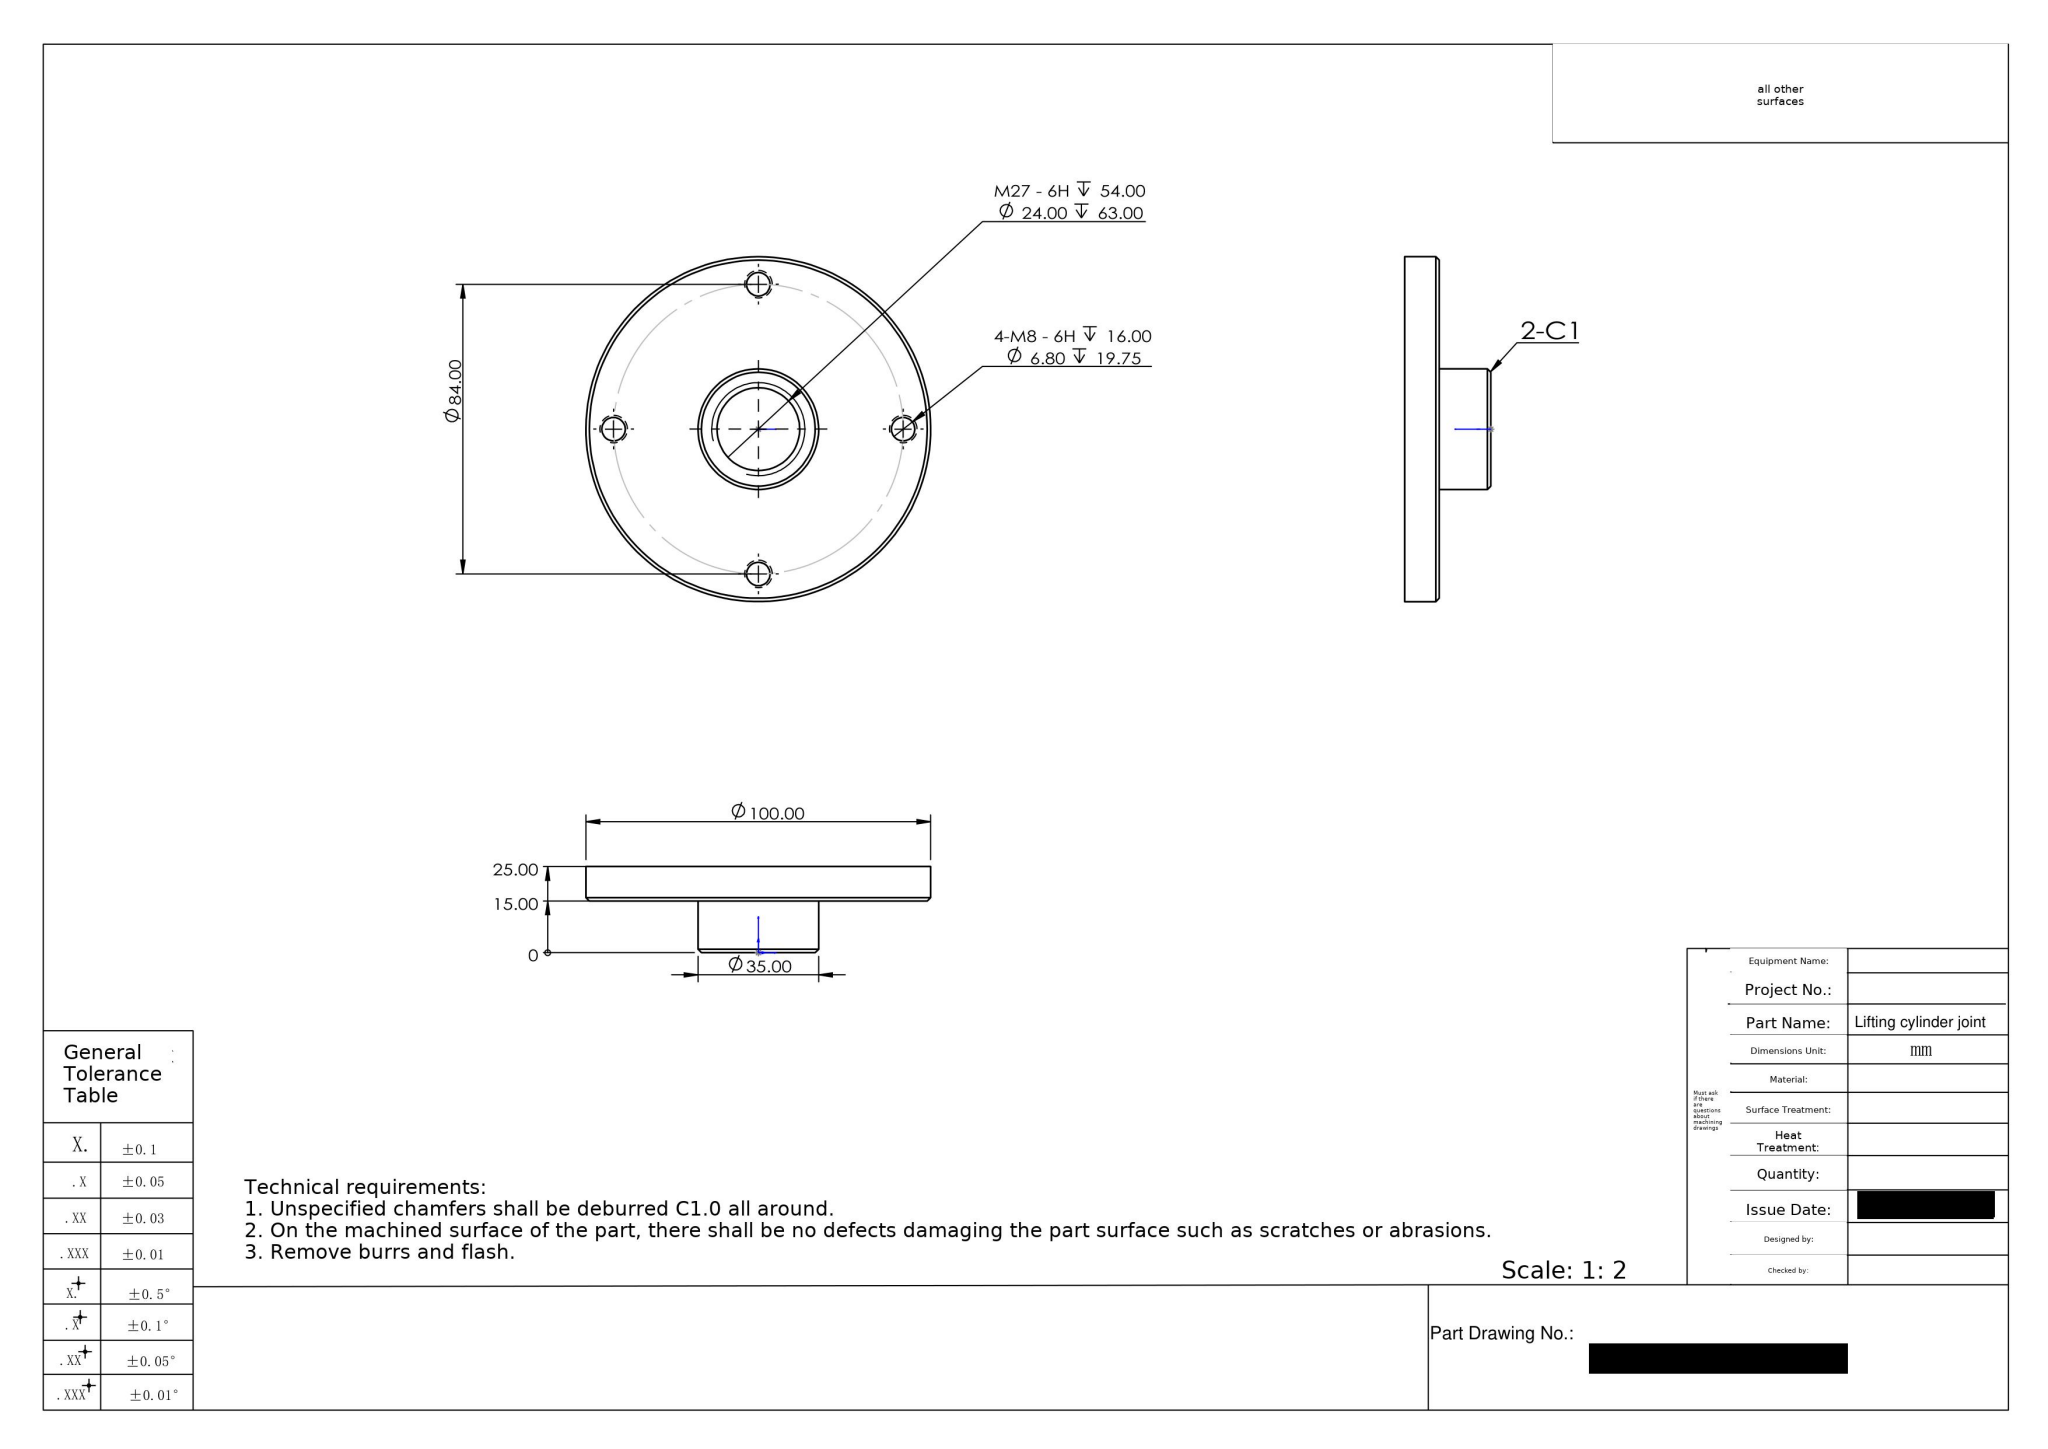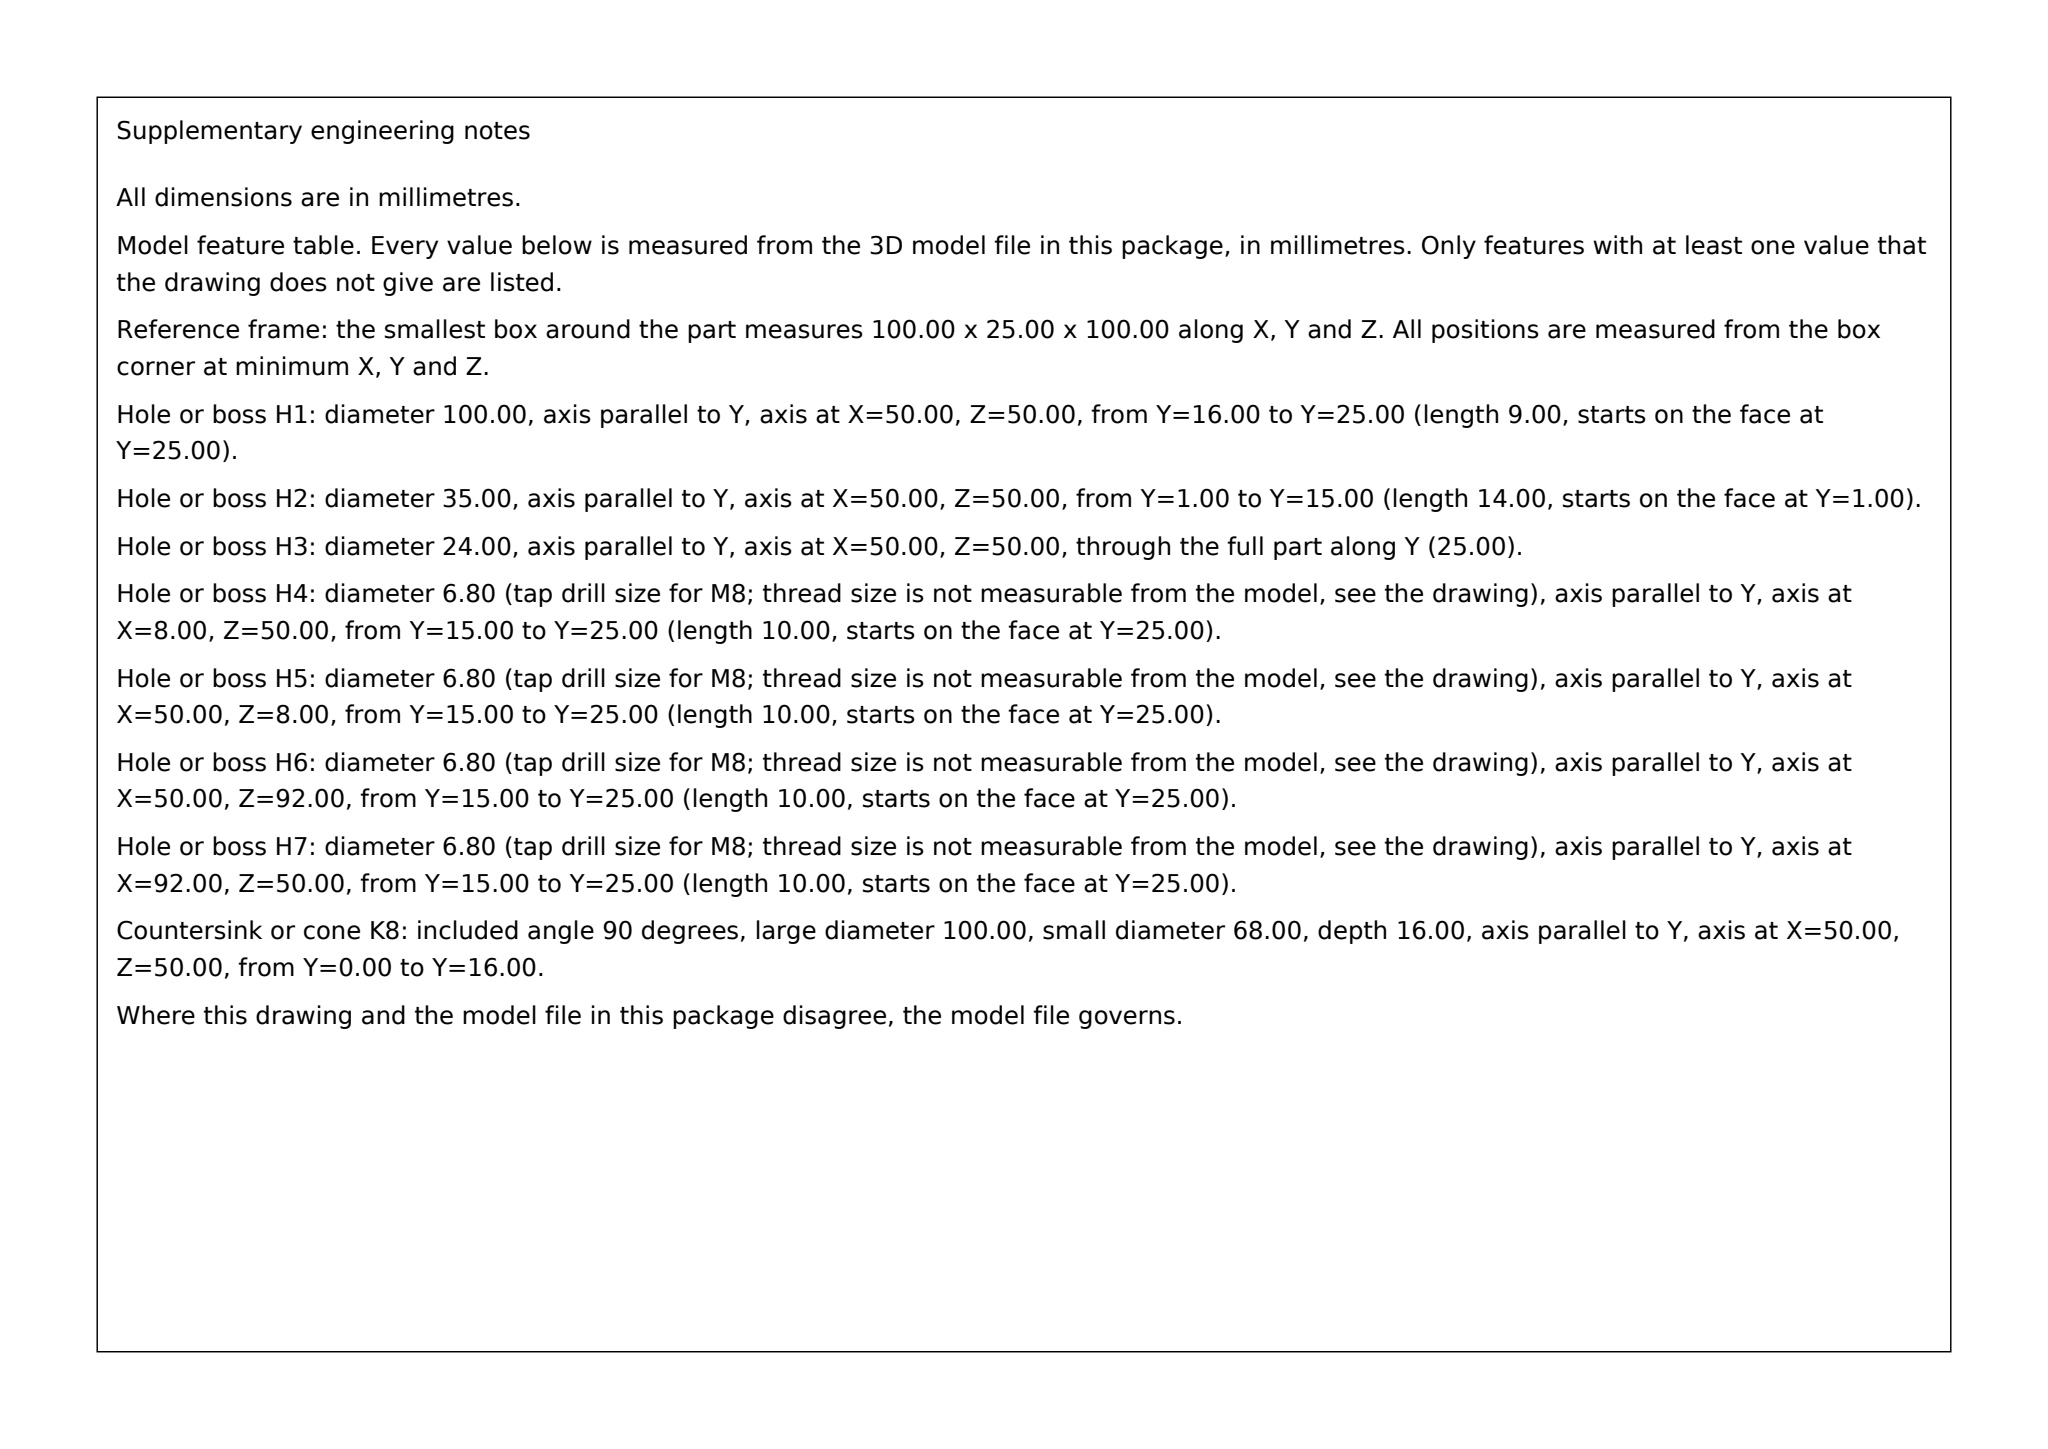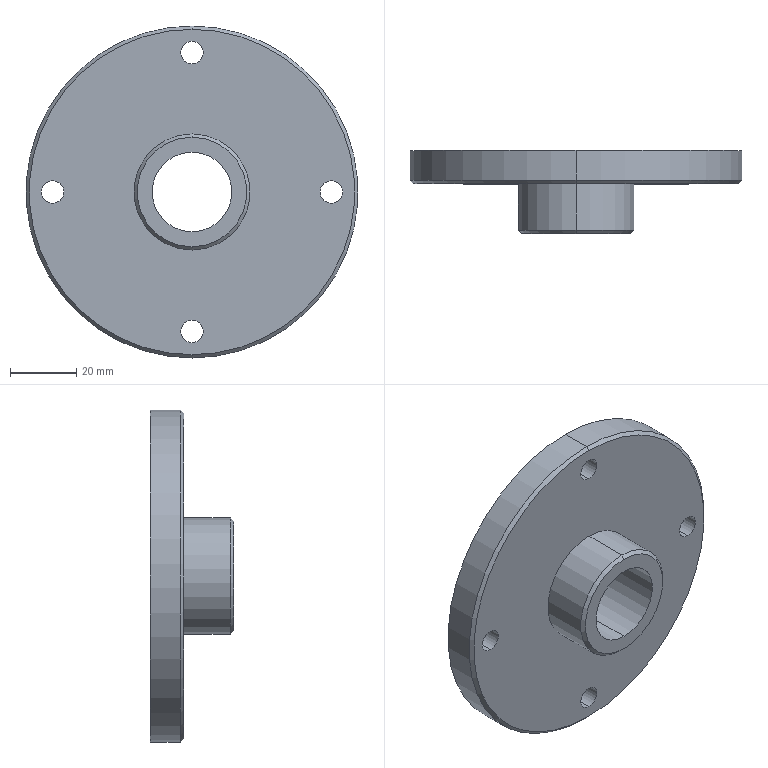Part | SolidWorks | mm | 1 solid | 21 faces | box 100 x 25 x 100 mm | volume 79999 mm3 | cylinder 14 | cone 4 | plane 3 | commonest cylinder face diameters 6.8 x8 24 x2 100 x2 35 x2
build123d program:
from build123d import *

# Parameters (mm, degrees)
SKETCH1_R              = 17.5
BOSS_EXTRUDE1_DEPTH    = 15
SKETCH2_R              = 50
BOSS_EXTRUDE2_DEPTH    = 10
M27_TAPPED_HOLE1_D     = 24
M27_TAPPED_HOLE1_DEPTH = 63
M27_TAPPED_HOLE1_TIP   = 7.21
M8_TAPPED_HOLE1_D      = 6.8
M8_TAPPED_HOLE1_DEPTH  = 19.75
M8_TAPPED_HOLE1_TIP    = 2.043
CHAMFER1_SIZE          = 1


with BuildPart() as part:
    # Sketch1 → Boss-Extrude1 (new body)
    with BuildSketch(Plane(origin=(0, 0, 0), x_dir=(1, 0, 0), z_dir=(0, 1, 0))):
        with Locations(Location((0, 0, 0), (0, 0, 270))):
            Circle(SKETCH1_R)
    extrude(amount=BOSS_EXTRUDE1_DEPTH)

    # Sketch2 → Boss-Extrude2 (add)
    with BuildSketch(Plane(origin=(0, 15, 0), x_dir=(1, 0, 0), z_dir=(0, 1, 0))):
        with Locations(Location((0, 0, 0), (0, 0, 270))):
            Circle(SKETCH2_R)
    extrude(amount=BOSS_EXTRUDE2_DEPTH)

    # M27 Tapped Hole1
    with Locations(Plane(origin=(0, 0, 0), x_dir=(-1, 0, 0), z_dir=(0, -1, 0))):
        with Locations((0, 0)):
            Hole(M27_TAPPED_HOLE1_D / 2, depth=M27_TAPPED_HOLE1_DEPTH)
            with Locations((0, 0, -(M27_TAPPED_HOLE1_DEPTH + M27_TAPPED_HOLE1_TIP / 2))):  # 118° drill point
                Cone(0, M27_TAPPED_HOLE1_D / 2, M27_TAPPED_HOLE1_TIP, mode=Mode.SUBTRACT)

    # M8 Tapped Hole1
    with Locations(Plane(origin=(0, 25, 0), x_dir=(1, 0, 0), z_dir=(0, 1, 0))):
        with Locations((0, 42), (42, 0), (0, -42), (-42, 0)):
            Hole(M8_TAPPED_HOLE1_D / 2, depth=M8_TAPPED_HOLE1_DEPTH)
            with Locations((0, 0, -(M8_TAPPED_HOLE1_DEPTH + M8_TAPPED_HOLE1_TIP / 2))):  # 118° drill point
                Cone(0, M8_TAPPED_HOLE1_D / 2, M8_TAPPED_HOLE1_TIP, mode=Mode.SUBTRACT)

    # Chamfer1
    chamfer1_edges = [part.edges().sort_by_distance(p)[0] for p in [
        (0, 0, -17.5),
        (0, 15, -50),
    ]]
    chamfer(chamfer1_edges, length=CHAMFER1_SIZE)


solid = part.part
STEP:
#1=CARTESIAN_POINT('',(0.,15.,-49.));
#2=VERTEX_POINT('',#1);
#3=CARTESIAN_POINT('',(0.,15.,49.));
#4=VERTEX_POINT('',#3);
#5=CARTESIAN_POINT('',(0.,15.,0.));
#6=DIRECTION('',(0.,-1.,0.));
#7=DIRECTION('',(0.,0.,1.));
#8=AXIS2_PLACEMENT_3D('',#5,#6,#7);
#9=CIRCLE('',#8,49.);
#10=EDGE_CURVE('',#2,#4,#9,.T.);
#11=ORIENTED_EDGE('',*,*,#10,.F.);
#12=CARTESIAN_POINT('',(0.,16.,-50.));
#13=VERTEX_POINT('',#12);
#14=CARTESIAN_POINT('',(0.,16.,-50.));
#15=DIRECTION('',(0.,0.7071,-0.7071));
#16=VECTOR('',#15,1000.);
#17=LINE('',#14,#16);
#18=EDGE_CURVE('',#2,#13,#17,.T.);
#19=ORIENTED_EDGE('',*,*,#18,.T.);
#20=CARTESIAN_POINT('',(0.,16.,50.));
#21=VERTEX_POINT('',#20);
#22=CARTESIAN_POINT('',(0.,16.,0.));
#23=DIRECTION('',(0.,1.,0.));
#24=DIRECTION('',(0.,0.,1.));
#25=AXIS2_PLACEMENT_3D('',#22,#23,#24);
#26=CIRCLE('',#25,50.);
#27=EDGE_CURVE('',#21,#13,#26,.T.);
#28=ORIENTED_EDGE('',*,*,#27,.F.);
#29=CARTESIAN_POINT('',(0.,16.,50.));
#30=DIRECTION('',(0.,0.7071,0.7071));
#31=VECTOR('',#30,1000.);
#32=LINE('',#29,#31);
#33=EDGE_CURVE('',#4,#21,#32,.T.);
#34=ORIENTED_EDGE('',*,*,#33,.F.);
#35=EDGE_LOOP('',(#11,#19,#28,#34));
#36=FACE_OUTER_BOUND('',#35,.T.);
#37=CARTESIAN_POINT('',(0.,16.,0.));
#38=DIRECTION('',(0.,1.,0.));
#39=DIRECTION('',(0.,0.,1.));
#40=AXIS2_PLACEMENT_3D('',#37,#38,#39);
#41=CONICAL_SURFACE('',#40,50.,0.7854);
#42=ADVANCED_FACE('',(#36),#41,.T.);
#43=CARTESIAN_POINT('',(0.,0.,-16.5));
#44=VERTEX_POINT('',#43);
#45=CARTESIAN_POINT('',(0.,0.,16.5));
#46=VERTEX_POINT('',#45);
#47=CARTESIAN_POINT('',(0.,0.,0.));
#48=DIRECTION('',(0.,-1.,0.));
#49=DIRECTION('',(0.,0.,1.));
#50=AXIS2_PLACEMENT_3D('',#47,#48,#49);
#51=CIRCLE('',#50,16.5);
#52=EDGE_CURVE('',#44,#46,#51,.T.);
#53=ORIENTED_EDGE('',*,*,#52,.F.);
#54=CARTESIAN_POINT('',(0.,1.,-17.5));
#55=VERTEX_POINT('',#54);
#56=CARTESIAN_POINT('',(0.,1.,-17.5));
#57=DIRECTION('',(0.,0.7071,-0.7071));
#58=VECTOR('',#57,1000.);
#59=LINE('',#56,#58);
#60=EDGE_CURVE('',#44,#55,#59,.T.);
#61=ORIENTED_EDGE('',*,*,#60,.T.);
#62=CARTESIAN_POINT('',(0.,1.,17.5));
#63=VERTEX_POINT('',#62);
#64=CARTESIAN_POINT('',(0.,1.,0.));
#65=DIRECTION('',(0.,1.,0.));
#66=DIRECTION('',(0.,0.,1.));
#67=AXIS2_PLACEMENT_3D('',#64,#65,#66);
#68=CIRCLE('',#67,17.5);
#69=EDGE_CURVE('',#63,#55,#68,.T.);
#70=ORIENTED_EDGE('',*,*,#69,.F.);
#71=CARTESIAN_POINT('',(0.,1.,17.5));
#72=DIRECTION('',(0.,0.7071,0.7071));
#73=VECTOR('',#72,1000.);
#74=LINE('',#71,#73);
#75=EDGE_CURVE('',#46,#63,#74,.T.);
#76=ORIENTED_EDGE('',*,*,#75,.F.);
#77=EDGE_LOOP('',(#53,#61,#70,#76));
#78=FACE_OUTER_BOUND('',#77,.T.);
#79=CARTESIAN_POINT('',(0.,1.,0.));
#80=DIRECTION('',(0.,1.,0.));
#81=DIRECTION('',(0.,0.,1.));
#82=AXIS2_PLACEMENT_3D('',#79,#80,#81);
#83=CONICAL_SURFACE('',#82,17.5,0.7854);
#84=ADVANCED_FACE('',(#78),#83,.T.);
#85=CARTESIAN_POINT('',(0.,15.,-45.4));
#86=VERTEX_POINT('',#85);
#87=CARTESIAN_POINT('',(0.,15.,-38.6));
#88=VERTEX_POINT('',#87);
#89=CARTESIAN_POINT('',(0.,15.,-42.));
#90=DIRECTION('',(0.,1.,0.));
#91=DIRECTION('',(0.,0.,1.));
#92=AXIS2_PLACEMENT_3D('',#89,#90,#91);
#93=CIRCLE('',#92,3.4);
#94=EDGE_CURVE('',#86,#88,#93,.T.);
#95=ORIENTED_EDGE('',*,*,#94,.F.);
#96=CARTESIAN_POINT('',(0.,25.,-45.4));
#97=VERTEX_POINT('',#96);
#98=CARTESIAN_POINT('',(0.,25.,-45.4));
#99=DIRECTION('',(0.,1.,0.));
#100=VECTOR('',#99,1000.);
#101=LINE('',#98,#100);
#102=EDGE_CURVE('',#86,#97,#101,.T.);
#103=ORIENTED_EDGE('',*,*,#102,.T.);
#104=CARTESIAN_POINT('',(0.,25.,-38.6));
#105=VERTEX_POINT('',#104);
#106=CARTESIAN_POINT('',(0.,25.,-42.));
#107=DIRECTION('',(0.,1.,0.));
#108=DIRECTION('',(0.,0.,1.));
#109=AXIS2_PLACEMENT_3D('',#106,#107,#108);
#110=CIRCLE('',#109,3.4);
#111=EDGE_CURVE('',#97,#105,#110,.T.);
#112=ORIENTED_EDGE('',*,*,#111,.T.);
#113=CARTESIAN_POINT('',(0.,25.,-38.6));
#114=DIRECTION('',(0.,1.,0.));
#115=VECTOR('',#114,1000.);
#116=LINE('',#113,#115);
#117=EDGE_CURVE('',#88,#105,#116,.T.);
#118=ORIENTED_EDGE('',*,*,#117,.F.);
#119=EDGE_LOOP('',(#95,#103,#112,#118));
#120=FACE_OUTER_BOUND('',#119,.T.);
#121=CARTESIAN_POINT('',(0.,25.,-42.));
#122=DIRECTION('',(0.,1.,0.));
#123=DIRECTION('',(0.,0.,1.));
#124=AXIS2_PLACEMENT_3D('',#121,#122,#123);
#125=CYLINDRICAL_SURFACE('',#124,3.4);
#126=ADVANCED_FACE('',(#120),#125,.F.);
#127=CARTESIAN_POINT('',(42.,15.,-3.4));
#128=VERTEX_POINT('',#127);
#129=CARTESIAN_POINT('',(42.,15.,3.4));
#130=VERTEX_POINT('',#129);
#131=CARTESIAN_POINT('',(42.,15.,0.));
#132=DIRECTION('',(0.,1.,0.));
#133=DIRECTION('',(0.,0.,1.));
#134=AXIS2_PLACEMENT_3D('',#131,#132,#133);
#135=CIRCLE('',#134,3.4);
#136=EDGE_CURVE('',#128,#130,#135,.T.);
#137=ORIENTED_EDGE('',*,*,#136,.F.);
#138=CARTESIAN_POINT('',(42.,25.,-3.4));
#139=VERTEX_POINT('',#138);
#140=CARTESIAN_POINT('',(42.,25.,-3.4));
#141=DIRECTION('',(0.,1.,0.));
#142=VECTOR('',#141,1000.);
#143=LINE('',#140,#142);
#144=EDGE_CURVE('',#128,#139,#143,.T.);
#145=ORIENTED_EDGE('',*,*,#144,.T.);
#146=CARTESIAN_POINT('',(42.,25.,3.4));
#147=VERTEX_POINT('',#146);
#148=CARTESIAN_POINT('',(42.,25.,0.));
#149=DIRECTION('',(0.,1.,0.));
#150=DIRECTION('',(0.,0.,1.));
#151=AXIS2_PLACEMENT_3D('',#148,#149,#150);
#152=CIRCLE('',#151,3.4);
#153=EDGE_CURVE('',#139,#147,#152,.T.);
#154=ORIENTED_EDGE('',*,*,#153,.T.);
#155=CARTESIAN_POINT('',(42.,25.,3.4));
#156=DIRECTION('',(0.,1.,0.));
#157=VECTOR('',#156,1000.);
#158=LINE('',#155,#157);
#159=EDGE_CURVE('',#130,#147,#158,.T.);
#160=ORIENTED_EDGE('',*,*,#159,.F.);
#161=EDGE_LOOP('',(#137,#145,#154,#160));
#162=FACE_OUTER_BOUND('',#161,.T.);
#163=CARTESIAN_POINT('',(42.,25.,0.));
#164=DIRECTION('',(0.,1.,0.));
#165=DIRECTION('',(0.,0.,1.));
#166=AXIS2_PLACEMENT_3D('',#163,#164,#165);
#167=CYLINDRICAL_SURFACE('',#166,3.4);
#168=ADVANCED_FACE('',(#162),#167,.F.);
#169=CARTESIAN_POINT('',(0.,15.,38.6));
#170=VERTEX_POINT('',#169);
#171=CARTESIAN_POINT('',(0.,15.,45.4));
#172=VERTEX_POINT('',#171);
#173=CARTESIAN_POINT('',(0.,15.,42.));
#174=DIRECTION('',(0.,1.,0.));
#175=DIRECTION('',(0.,0.,1.));
#176=AXIS2_PLACEMENT_3D('',#173,#174,#175);
#177=CIRCLE('',#176,3.4);
#178=EDGE_CURVE('',#170,#172,#177,.T.);
#179=ORIENTED_EDGE('',*,*,#178,.F.);
#180=CARTESIAN_POINT('',(0.,25.,38.6));
#181=VERTEX_POINT('',#180);
#182=CARTESIAN_POINT('',(0.,25.,38.6));
#183=DIRECTION('',(0.,1.,0.));
#184=VECTOR('',#183,1000.);
#185=LINE('',#182,#184);
#186=EDGE_CURVE('',#170,#181,#185,.T.);
#187=ORIENTED_EDGE('',*,*,#186,.T.);
#188=CARTESIAN_POINT('',(0.,25.,45.4));
#189=VERTEX_POINT('',#188);
#190=CARTESIAN_POINT('',(0.,25.,42.));
#191=DIRECTION('',(0.,1.,0.));
#192=DIRECTION('',(0.,0.,1.));
#193=AXIS2_PLACEMENT_3D('',#190,#191,#192);
#194=CIRCLE('',#193,3.4);
#195=EDGE_CURVE('',#181,#189,#194,.T.);
#196=ORIENTED_EDGE('',*,*,#195,.T.);
#197=CARTESIAN_POINT('',(0.,25.,45.4));
#198=DIRECTION('',(0.,1.,0.));
#199=VECTOR('',#198,1000.);
#200=LINE('',#197,#199);
#201=EDGE_CURVE('',#172,#189,#200,.T.);
#202=ORIENTED_EDGE('',*,*,#201,.F.);
#203=EDGE_LOOP('',(#179,#187,#196,#202));
#204=FACE_OUTER_BOUND('',#203,.T.);
#205=CARTESIAN_POINT('',(0.,25.,42.));
#206=DIRECTION('',(0.,1.,0.));
#207=DIRECTION('',(0.,0.,1.));
#208=AXIS2_PLACEMENT_3D('',#205,#206,#207);
#209=CYLINDRICAL_SURFACE('',#208,3.4);
#210=ADVANCED_FACE('',(#204),#209,.F.);
#211=CARTESIAN_POINT('',(-42.,15.,-3.4));
#212=VERTEX_POINT('',#211);
#213=CARTESIAN_POINT('',(-42.,15.,3.4));
#214=VERTEX_POINT('',#213);
#215=CARTESIAN_POINT('',(-42.,15.,0.));
#216=DIRECTION('',(0.,1.,0.));
#217=DIRECTION('',(0.,0.,1.));
#218=AXIS2_PLACEMENT_3D('',#215,#216,#217);
#219=CIRCLE('',#218,3.4);
#220=EDGE_CURVE('',#212,#214,#219,.T.);
#221=ORIENTED_EDGE('',*,*,#220,.F.);
#222=CARTESIAN_POINT('',(-42.,25.,-3.4));
#223=VERTEX_POINT('',#222);
#224=CARTESIAN_POINT('',(-42.,25.,-3.4));
#225=DIRECTION('',(0.,1.,0.));
#226=VECTOR('',#225,1000.);
#227=LINE('',#224,#226);
#228=EDGE_CURVE('',#212,#223,#227,.T.);
#229=ORIENTED_EDGE('',*,*,#228,.T.);
#230=CARTESIAN_POINT('',(-42.,25.,3.4));
#231=VERTEX_POINT('',#230);
#232=CARTESIAN_POINT('',(-42.,25.,0.));
#233=DIRECTION('',(0.,1.,0.));
#234=DIRECTION('',(0.,0.,1.));
#235=AXIS2_PLACEMENT_3D('',#232,#233,#234);
#236=CIRCLE('',#235,3.4);
#237=EDGE_CURVE('',#223,#231,#236,.T.);
#238=ORIENTED_EDGE('',*,*,#237,.T.);
#239=CARTESIAN_POINT('',(-42.,25.,3.4));
#240=DIRECTION('',(0.,1.,0.));
#241=VECTOR('',#240,1000.);
#242=LINE('',#239,#241);
#243=EDGE_CURVE('',#214,#231,#242,.T.);
#244=ORIENTED_EDGE('',*,*,#243,.F.);
#245=EDGE_LOOP('',(#221,#229,#238,#244));
#246=FACE_OUTER_BOUND('',#245,.T.);
#247=CARTESIAN_POINT('',(-42.,25.,0.));
#248=DIRECTION('',(0.,1.,0.));
#249=DIRECTION('',(0.,0.,1.));
#250=AXIS2_PLACEMENT_3D('',#247,#248,#249);
#251=CYLINDRICAL_SURFACE('',#250,3.4);
#252=ADVANCED_FACE('',(#246),#251,.F.);
#253=CARTESIAN_POINT('',(0.,25.,-12.));
#254=VERTEX_POINT('',#253);
#255=CARTESIAN_POINT('',(0.,25.,12.));
#256=VERTEX_POINT('',#255);
#257=CARTESIAN_POINT('',(0.,25.,0.));
#258=DIRECTION('',(0.,1.,0.));
#259=DIRECTION('',(0.,0.,1.));
#260=AXIS2_PLACEMENT_3D('',#257,#258,#259);
#261=CIRCLE('',#260,12.);
#262=EDGE_CURVE('',#254,#256,#261,.T.);
#263=ORIENTED_EDGE('',*,*,#262,.T.);
#264=CARTESIAN_POINT('',(0.,0.,12.));
#265=VERTEX_POINT('',#264);
#266=CARTESIAN_POINT('',(0.,0.,12.));
#267=DIRECTION('',(0.,-1.,0.));
#268=VECTOR('',#267,1000.);
#269=LINE('',#266,#268);
#270=EDGE_CURVE('',#256,#265,#269,.T.);
#271=ORIENTED_EDGE('',*,*,#270,.T.);
#272=CARTESIAN_POINT('',(0.,0.,-12.));
#273=VERTEX_POINT('',#272);
#274=CARTESIAN_POINT('',(0.,0.,0.));
#275=DIRECTION('',(0.,-1.,0.));
#276=DIRECTION('',(0.,0.,-1.));
#277=AXIS2_PLACEMENT_3D('',#274,#275,#276);
#278=CIRCLE('',#277,12.);
#279=EDGE_CURVE('',#265,#273,#278,.T.);
#280=ORIENTED_EDGE('',*,*,#279,.T.);
#281=CARTESIAN_POINT('',(0.,0.,-12.));
#282=DIRECTION('',(0.,-1.,0.));
#283=VECTOR('',#282,1000.);
#284=LINE('',#281,#283);
#285=EDGE_CURVE('',#254,#273,#284,.T.);
#286=ORIENTED_EDGE('',*,*,#285,.F.);
#287=EDGE_LOOP('',(#263,#271,#280,#286));
#288=FACE_OUTER_BOUND('',#287,.T.);
#289=CARTESIAN_POINT('',(0.,0.,0.));
#290=DIRECTION('',(0.,-1.,0.));
#291=DIRECTION('',(0.,0.,-1.));
#292=AXIS2_PLACEMENT_3D('',#289,#290,#291);
#293=CYLINDRICAL_SURFACE('',#292,12.);
#294=ADVANCED_FACE('',(#288),#293,.F.);
#295=CARTESIAN_POINT('',(0.,25.,50.));
#296=VERTEX_POINT('',#295);
#297=CARTESIAN_POINT('',(0.,25.,-50.));
#298=VERTEX_POINT('',#297);
#299=CARTESIAN_POINT('',(0.,25.,0.));
#300=DIRECTION('',(0.,1.,0.));
#301=DIRECTION('',(0.,0.,1.));
#302=AXIS2_PLACEMENT_3D('',#299,#300,#301);
#303=CIRCLE('',#302,50.);
#304=EDGE_CURVE('',#296,#298,#303,.T.);
#305=ORIENTED_EDGE('',*,*,#304,.F.);
#306=CARTESIAN_POINT('',(0.,25.,50.));
#307=DIRECTION('',(0.,-1.,0.));
#308=VECTOR('',#307,1000.);
#309=LINE('',#306,#308);
#310=EDGE_CURVE('',#296,#21,#309,.T.);
#311=ORIENTED_EDGE('',*,*,#310,.T.);
#312=ORIENTED_EDGE('',*,*,#27,.T.);
#313=CARTESIAN_POINT('',(0.,25.,-50.));
#314=DIRECTION('',(0.,-1.,0.));
#315=VECTOR('',#314,1000.);
#316=LINE('',#313,#315);
#317=EDGE_CURVE('',#298,#13,#316,.T.);
#318=ORIENTED_EDGE('',*,*,#317,.F.);
#319=EDGE_LOOP('',(#305,#311,#312,#318));
#320=FACE_OUTER_BOUND('',#319,.T.);
#321=CARTESIAN_POINT('',(0.,25.,0.));
#322=DIRECTION('',(0.,-1.,0.));
#323=DIRECTION('',(0.,0.,-1.));
#324=AXIS2_PLACEMENT_3D('',#321,#322,#323);
#325=CYLINDRICAL_SURFACE('',#324,50.);
#326=ADVANCED_FACE('',(#320),#325,.T.);
#327=CARTESIAN_POINT('',(0.,15.,17.5));
#328=VERTEX_POINT('',#327);
#329=CARTESIAN_POINT('',(0.,15.,-17.5));
#330=VERTEX_POINT('',#329);
#331=CARTESIAN_POINT('',(0.,15.,0.));
#332=DIRECTION('',(0.,1.,0.));
#333=DIRECTION('',(0.,0.,1.));
#334=AXIS2_PLACEMENT_3D('',#331,#332,#333);
#335=CIRCLE('',#334,17.5);
#336=EDGE_CURVE('',#328,#330,#335,.T.);
#337=ORIENTED_EDGE('',*,*,#336,.F.);
#338=CARTESIAN_POINT('',(0.,15.,17.5));
#339=DIRECTION('',(0.,-1.,0.));
#340=VECTOR('',#339,1000.);
#341=LINE('',#338,#340);
#342=EDGE_CURVE('',#328,#63,#341,.T.);
#343=ORIENTED_EDGE('',*,*,#342,.T.);
#344=ORIENTED_EDGE('',*,*,#69,.T.);
#345=CARTESIAN_POINT('',(0.,15.,-17.5));
#346=DIRECTION('',(0.,-1.,0.));
#347=VECTOR('',#346,1000.);
#348=LINE('',#345,#347);
#349=EDGE_CURVE('',#330,#55,#348,.T.);
#350=ORIENTED_EDGE('',*,*,#349,.F.);
#351=EDGE_LOOP('',(#337,#343,#344,#350));
#352=FACE_OUTER_BOUND('',#351,.T.);
#353=CARTESIAN_POINT('',(0.,15.,0.));
#354=DIRECTION('',(0.,-1.,0.));
#355=DIRECTION('',(0.,0.,-1.));
#356=AXIS2_PLACEMENT_3D('',#353,#354,#355);
#357=CYLINDRICAL_SURFACE('',#356,17.5);
#358=ADVANCED_FACE('',(#352),#357,.T.);
#359=ORIENTED_EDGE('',*,*,#342,.F.);
#360=CARTESIAN_POINT('',(0.,15.,0.));
#361=DIRECTION('',(0.,1.,0.));
#362=DIRECTION('',(0.,0.,1.));
#363=AXIS2_PLACEMENT_3D('',#360,#361,#362);
#364=CIRCLE('',#363,17.5);
#365=EDGE_CURVE('',#330,#328,#364,.T.);
#366=ORIENTED_EDGE('',*,*,#365,.F.);
#367=ORIENTED_EDGE('',*,*,#349,.T.);
#368=CARTESIAN_POINT('',(0.,1.,0.));
#369=DIRECTION('',(0.,1.,0.));
#370=DIRECTION('',(0.,0.,1.));
#371=AXIS2_PLACEMENT_3D('',#368,#369,#370);
#372=CIRCLE('',#371,17.5);
#373=EDGE_CURVE('',#55,#63,#372,.T.);
#374=ORIENTED_EDGE('',*,*,#373,.T.);
#375=EDGE_LOOP('',(#359,#366,#367,#374));
#376=FACE_OUTER_BOUND('',#375,.T.);
#377=CARTESIAN_POINT('',(0.,15.,0.));
#378=DIRECTION('',(0.,-1.,0.));
#379=DIRECTION('',(0.,0.,-1.));
#380=AXIS2_PLACEMENT_3D('',#377,#378,#379);
#381=CYLINDRICAL_SURFACE('',#380,17.5);
#382=ADVANCED_FACE('',(#376),#381,.T.);
#383=CARTESIAN_POINT('',(0.,0.,0.));
#384=DIRECTION('',(0.,-1.,0.));
#385=DIRECTION('',(0.,0.,1.));
#386=AXIS2_PLACEMENT_3D('',#383,#384,#385);
#387=CIRCLE('',#386,16.5);
#388=EDGE_CURVE('',#46,#44,#387,.T.);
#389=ORIENTED_EDGE('',*,*,#388,.T.);
#390=ORIENTED_EDGE('',*,*,#52,.T.);
#391=EDGE_LOOP('',(#389,#390));
#392=FACE_OUTER_BOUND('',#391,.T.);
#393=CARTESIAN_POINT('',(0.,0.,0.));
#394=DIRECTION('',(0.,-1.,0.));
#395=DIRECTION('',(0.,0.,-1.));
#396=AXIS2_PLACEMENT_3D('',#393,#394,#395);
#397=CIRCLE('',#396,12.);
#398=EDGE_CURVE('',#273,#265,#397,.T.);
#399=ORIENTED_EDGE('',*,*,#398,.F.);
#400=ORIENTED_EDGE('',*,*,#279,.F.);
#401=EDGE_LOOP('',(#399,#400));
#402=FACE_BOUND('',#401,.T.);
#403=CARTESIAN_POINT('',(0.,0.,0.));
#404=DIRECTION('',(0.,1.,0.));
#405=DIRECTION('',(0.,0.,1.));
#406=AXIS2_PLACEMENT_3D('',#403,#404,#405);
#407=PLANE('',#406);
#408=ADVANCED_FACE('',(#392,#402),#407,.F.);
#409=CARTESIAN_POINT('',(0.,15.,0.));
#410=DIRECTION('',(0.,-1.,0.));
#411=DIRECTION('',(0.,0.,1.));
#412=AXIS2_PLACEMENT_3D('',#409,#410,#411);
#413=CIRCLE('',#412,49.);
#414=EDGE_CURVE('',#4,#2,#413,.T.);
#415=ORIENTED_EDGE('',*,*,#414,.T.);
#416=ORIENTED_EDGE('',*,*,#10,.T.);
#417=EDGE_LOOP('',(#415,#416));
#418=FACE_OUTER_BOUND('',#417,.T.);
#419=CARTESIAN_POINT('',(0.,15.,-42.));
#420=DIRECTION('',(0.,1.,0.));
#421=DIRECTION('',(0.,0.,1.));
#422=AXIS2_PLACEMENT_3D('',#419,#420,#421);
#423=CIRCLE('',#422,3.4);
#424=EDGE_CURVE('',#88,#86,#423,.T.);
#425=ORIENTED_EDGE('',*,*,#424,.T.);
#426=ORIENTED_EDGE('',*,*,#94,.T.);
#427=EDGE_LOOP('',(#425,#426));
#428=FACE_BOUND('',#427,.T.);
#429=CARTESIAN_POINT('',(42.,15.,0.));
#430=DIRECTION('',(0.,1.,0.));
#431=DIRECTION('',(0.,0.,1.));
#432=AXIS2_PLACEMENT_3D('',#429,#430,#431);
#433=CIRCLE('',#432,3.4);
#434=EDGE_CURVE('',#130,#128,#433,.T.);
#435=ORIENTED_EDGE('',*,*,#434,.T.);
#436=ORIENTED_EDGE('',*,*,#136,.T.);
#437=EDGE_LOOP('',(#435,#436));
#438=FACE_BOUND('',#437,.T.);
#439=CARTESIAN_POINT('',(0.,15.,42.));
#440=DIRECTION('',(0.,1.,0.));
#441=DIRECTION('',(0.,0.,1.));
#442=AXIS2_PLACEMENT_3D('',#439,#440,#441);
#443=CIRCLE('',#442,3.4);
#444=EDGE_CURVE('',#172,#170,#443,.T.);
#445=ORIENTED_EDGE('',*,*,#444,.T.);
#446=ORIENTED_EDGE('',*,*,#178,.T.);
#447=EDGE_LOOP('',(#445,#446));
#448=FACE_BOUND('',#447,.T.);
#449=CARTESIAN_POINT('',(-42.,15.,0.));
#450=DIRECTION('',(0.,1.,0.));
#451=DIRECTION('',(0.,0.,1.));
#452=AXIS2_PLACEMENT_3D('',#449,#450,#451);
#453=CIRCLE('',#452,3.4);
#454=EDGE_CURVE('',#214,#212,#453,.T.);
#455=ORIENTED_EDGE('',*,*,#454,.T.);
#456=ORIENTED_EDGE('',*,*,#220,.T.);
#457=EDGE_LOOP('',(#455,#456));
#458=FACE_BOUND('',#457,.T.);
#459=ORIENTED_EDGE('',*,*,#365,.T.);
#460=ORIENTED_EDGE('',*,*,#336,.T.);
#461=EDGE_LOOP('',(#459,#460));
#462=FACE_BOUND('',#461,.T.);
#463=CARTESIAN_POINT('',(0.,15.,0.));
#464=DIRECTION('',(0.,1.,0.));
#465=DIRECTION('',(0.,0.,1.));
#466=AXIS2_PLACEMENT_3D('',#463,#464,#465);
#467=PLANE('',#466);
#468=ADVANCED_FACE('',(#418,#428,#438,#448,#458,#462),#467,.F.);
#469=ORIENTED_EDGE('',*,*,#310,.F.);
#470=CARTESIAN_POINT('',(0.,25.,0.));
#471=DIRECTION('',(0.,1.,0.));
#472=DIRECTION('',(0.,0.,1.));
#473=AXIS2_PLACEMENT_3D('',#470,#471,#472);
#474=CIRCLE('',#473,50.);
#475=EDGE_CURVE('',#298,#296,#474,.T.);
#476=ORIENTED_EDGE('',*,*,#475,.F.);
#477=ORIENTED_EDGE('',*,*,#317,.T.);
#478=CARTESIAN_POINT('',(0.,16.,0.));
#479=DIRECTION('',(0.,1.,0.));
#480=DIRECTION('',(0.,0.,1.));
#481=AXIS2_PLACEMENT_3D('',#478,#479,#480);
#482=CIRCLE('',#481,50.);
#483=EDGE_CURVE('',#13,#21,#482,.T.);
#484=ORIENTED_EDGE('',*,*,#483,.T.);
#485=EDGE_LOOP('',(#469,#476,#477,#484));
#486=FACE_OUTER_BOUND('',#485,.T.);
#487=CARTESIAN_POINT('',(0.,25.,0.));
#488=DIRECTION('',(0.,-1.,0.));
#489=DIRECTION('',(0.,0.,-1.));
#490=AXIS2_PLACEMENT_3D('',#487,#488,#489);
#491=CYLINDRICAL_SURFACE('',#490,50.);
#492=ADVANCED_FACE('',(#486),#491,.T.);
#493=CARTESIAN_POINT('',(0.,25.,-42.));
#494=DIRECTION('',(0.,1.,0.));
#495=DIRECTION('',(0.,0.,1.));
#496=AXIS2_PLACEMENT_3D('',#493,#494,#495);
#497=CIRCLE('',#496,3.4);
#498=EDGE_CURVE('',#105,#97,#497,.T.);
#499=ORIENTED_EDGE('',*,*,#498,.F.);
#500=ORIENTED_EDGE('',*,*,#111,.F.);
#501=EDGE_LOOP('',(#499,#500));
#502=FACE_BOUND('',#501,.T.);
#503=CARTESIAN_POINT('',(42.,25.,0.));
#504=DIRECTION('',(0.,1.,0.));
#505=DIRECTION('',(0.,0.,1.));
#506=AXIS2_PLACEMENT_3D('',#503,#504,#505);
#507=CIRCLE('',#506,3.4);
#508=EDGE_CURVE('',#147,#139,#507,.T.);
#509=ORIENTED_EDGE('',*,*,#508,.F.);
#510=ORIENTED_EDGE('',*,*,#153,.F.);
#511=EDGE_LOOP('',(#509,#510));
#512=FACE_BOUND('',#511,.T.);
#513=CARTESIAN_POINT('',(0.,25.,42.));
#514=DIRECTION('',(0.,1.,0.));
#515=DIRECTION('',(0.,0.,1.));
#516=AXIS2_PLACEMENT_3D('',#513,#514,#515);
#517=CIRCLE('',#516,3.4);
#518=EDGE_CURVE('',#189,#181,#517,.T.);
#519=ORIENTED_EDGE('',*,*,#518,.F.);
#520=ORIENTED_EDGE('',*,*,#195,.F.);
#521=EDGE_LOOP('',(#519,#520));
#522=FACE_BOUND('',#521,.T.);
#523=CARTESIAN_POINT('',(-42.,25.,0.));
#524=DIRECTION('',(0.,1.,0.));
#525=DIRECTION('',(0.,0.,1.));
#526=AXIS2_PLACEMENT_3D('',#523,#524,#525);
#527=CIRCLE('',#526,3.4);
#528=EDGE_CURVE('',#231,#223,#527,.T.);
#529=ORIENTED_EDGE('',*,*,#528,.F.);
#530=ORIENTED_EDGE('',*,*,#237,.F.);
#531=EDGE_LOOP('',(#529,#530));
#532=FACE_BOUND('',#531,.T.);
#533=ORIENTED_EDGE('',*,*,#262,.F.);
#534=CARTESIAN_POINT('',(0.,25.,0.));
#535=DIRECTION('',(0.,1.,0.));
#536=DIRECTION('',(0.,0.,1.));
#537=AXIS2_PLACEMENT_3D('',#534,#535,#536);
#538=CIRCLE('',#537,12.);
#539=EDGE_CURVE('',#256,#254,#538,.T.);
#540=ORIENTED_EDGE('',*,*,#539,.F.);
#541=EDGE_LOOP('',(#533,#540));
#542=FACE_BOUND('',#541,.T.);
#543=ORIENTED_EDGE('',*,*,#475,.T.);
#544=ORIENTED_EDGE('',*,*,#304,.T.);
#545=EDGE_LOOP('',(#543,#544));
#546=FACE_OUTER_BOUND('',#545,.T.);
#547=CARTESIAN_POINT('',(0.,25.,0.));
#548=DIRECTION('',(0.,1.,0.));
#549=DIRECTION('',(0.,0.,1.));
#550=AXIS2_PLACEMENT_3D('',#547,#548,#549);
#551=PLANE('',#550);
#552=ADVANCED_FACE('',(#502,#512,#522,#532,#542,#546),#551,.T.);
#553=ORIENTED_EDGE('',*,*,#270,.F.);
#554=ORIENTED_EDGE('',*,*,#539,.T.);
#555=ORIENTED_EDGE('',*,*,#285,.T.);
#556=ORIENTED_EDGE('',*,*,#398,.T.);
#557=EDGE_LOOP('',(#553,#554,#555,#556));
#558=FACE_OUTER_BOUND('',#557,.T.);
#559=CARTESIAN_POINT('',(0.,0.,0.));
#560=DIRECTION('',(0.,-1.,0.));
#561=DIRECTION('',(0.,0.,-1.));
#562=AXIS2_PLACEMENT_3D('',#559,#560,#561);
#563=CYLINDRICAL_SURFACE('',#562,12.);
#564=ADVANCED_FACE('',(#558),#563,.F.);
#565=ORIENTED_EDGE('',*,*,#228,.F.);
#566=ORIENTED_EDGE('',*,*,#454,.F.);
#567=ORIENTED_EDGE('',*,*,#243,.T.);
#568=ORIENTED_EDGE('',*,*,#528,.T.);
#569=EDGE_LOOP('',(#565,#566,#567,#568));
#570=FACE_OUTER_BOUND('',#569,.T.);
#571=CARTESIAN_POINT('',(-42.,25.,0.));
#572=DIRECTION('',(0.,1.,0.));
#573=DIRECTION('',(0.,0.,1.));
#574=AXIS2_PLACEMENT_3D('',#571,#572,#573);
#575=CYLINDRICAL_SURFACE('',#574,3.4);
#576=ADVANCED_FACE('',(#570),#575,.F.);
#577=ORIENTED_EDGE('',*,*,#186,.F.);
#578=ORIENTED_EDGE('',*,*,#444,.F.);
#579=ORIENTED_EDGE('',*,*,#201,.T.);
#580=ORIENTED_EDGE('',*,*,#518,.T.);
#581=EDGE_LOOP('',(#577,#578,#579,#580));
#582=FACE_OUTER_BOUND('',#581,.T.);
#583=CARTESIAN_POINT('',(0.,25.,42.));
#584=DIRECTION('',(0.,1.,0.));
#585=DIRECTION('',(0.,0.,1.));
#586=AXIS2_PLACEMENT_3D('',#583,#584,#585);
#587=CYLINDRICAL_SURFACE('',#586,3.4);
#588=ADVANCED_FACE('',(#582),#587,.F.);
#589=ORIENTED_EDGE('',*,*,#144,.F.);
#590=ORIENTED_EDGE('',*,*,#434,.F.);
#591=ORIENTED_EDGE('',*,*,#159,.T.);
#592=ORIENTED_EDGE('',*,*,#508,.T.);
#593=EDGE_LOOP('',(#589,#590,#591,#592));
#594=FACE_OUTER_BOUND('',#593,.T.);
#595=CARTESIAN_POINT('',(42.,25.,0.));
#596=DIRECTION('',(0.,1.,0.));
#597=DIRECTION('',(0.,0.,1.));
#598=AXIS2_PLACEMENT_3D('',#595,#596,#597);
#599=CYLINDRICAL_SURFACE('',#598,3.4);
#600=ADVANCED_FACE('',(#594),#599,.F.);
#601=ORIENTED_EDGE('',*,*,#102,.F.);
#602=ORIENTED_EDGE('',*,*,#424,.F.);
#603=ORIENTED_EDGE('',*,*,#117,.T.);
#604=ORIENTED_EDGE('',*,*,#498,.T.);
#605=EDGE_LOOP('',(#601,#602,#603,#604));
#606=FACE_OUTER_BOUND('',#605,.T.);
#607=CARTESIAN_POINT('',(0.,25.,-42.));
#608=DIRECTION('',(0.,1.,0.));
#609=DIRECTION('',(0.,0.,1.));
#610=AXIS2_PLACEMENT_3D('',#607,#608,#609);
#611=CYLINDRICAL_SURFACE('',#610,3.4);
#612=ADVANCED_FACE('',(#606),#611,.F.);
#613=ORIENTED_EDGE('',*,*,#60,.F.);
#614=ORIENTED_EDGE('',*,*,#388,.F.);
#615=ORIENTED_EDGE('',*,*,#75,.T.);
#616=ORIENTED_EDGE('',*,*,#373,.F.);
#617=EDGE_LOOP('',(#613,#614,#615,#616));
#618=FACE_OUTER_BOUND('',#617,.T.);
#619=CARTESIAN_POINT('',(0.,1.,0.));
#620=DIRECTION('',(0.,1.,0.));
#621=DIRECTION('',(0.,0.,1.));
#622=AXIS2_PLACEMENT_3D('',#619,#620,#621);
#623=CONICAL_SURFACE('',#622,17.5,0.7854);
#624=ADVANCED_FACE('',(#618),#623,.T.);
#625=ORIENTED_EDGE('',*,*,#18,.F.);
#626=ORIENTED_EDGE('',*,*,#414,.F.);
#627=ORIENTED_EDGE('',*,*,#33,.T.);
#628=ORIENTED_EDGE('',*,*,#483,.F.);
#629=EDGE_LOOP('',(#625,#626,#627,#628));
#630=FACE_OUTER_BOUND('',#629,.T.);
#631=CARTESIAN_POINT('',(0.,16.,0.));
#632=DIRECTION('',(0.,1.,0.));
#633=DIRECTION('',(0.,0.,1.));
#634=AXIS2_PLACEMENT_3D('',#631,#632,#633);
#635=CONICAL_SURFACE('',#634,50.,0.7854);
#636=ADVANCED_FACE('',(#630),#635,.T.);
#637=CLOSED_SHELL('',(#42,#84,#126,#168,#210,#252,#294,#326,#358,#382,#408,#468,#492,#552,#564,#576,#588,#600,#612,#624,#636));
#638=MANIFOLD_SOLID_BREP('',#637);
#639=CARTESIAN_POINT('',(0.,0.,0.));
#640=DIRECTION('',(0.,0.,1.));
#641=DIRECTION('',(1.,0.,0.));
#642=AXIS2_PLACEMENT_3D('',#639,#640,#641);
#643=(LENGTH_UNIT()NAMED_UNIT(*)SI_UNIT(.MILLI.,.METRE.));
#644=UNCERTAINTY_MEASURE_WITH_UNIT(LENGTH_MEASURE(0.00001),#643,'','');
#645=(NAMED_UNIT(*)PLANE_ANGLE_UNIT()SI_UNIT($,.RADIAN.));
#646=(NAMED_UNIT(*)SI_UNIT($,.STERADIAN.)SOLID_ANGLE_UNIT());
#647=(GEOMETRIC_REPRESENTATION_CONTEXT(3)GLOBAL_UNCERTAINTY_ASSIGNED_CONTEXT((#644))GLOBAL_UNIT_ASSIGNED_CONTEXT((#643,#645,#646))REPRESENTATION_CONTEXT('',''));
#648=ADVANCED_BREP_SHAPE_REPRESENTATION('',(#638,#642),#647);